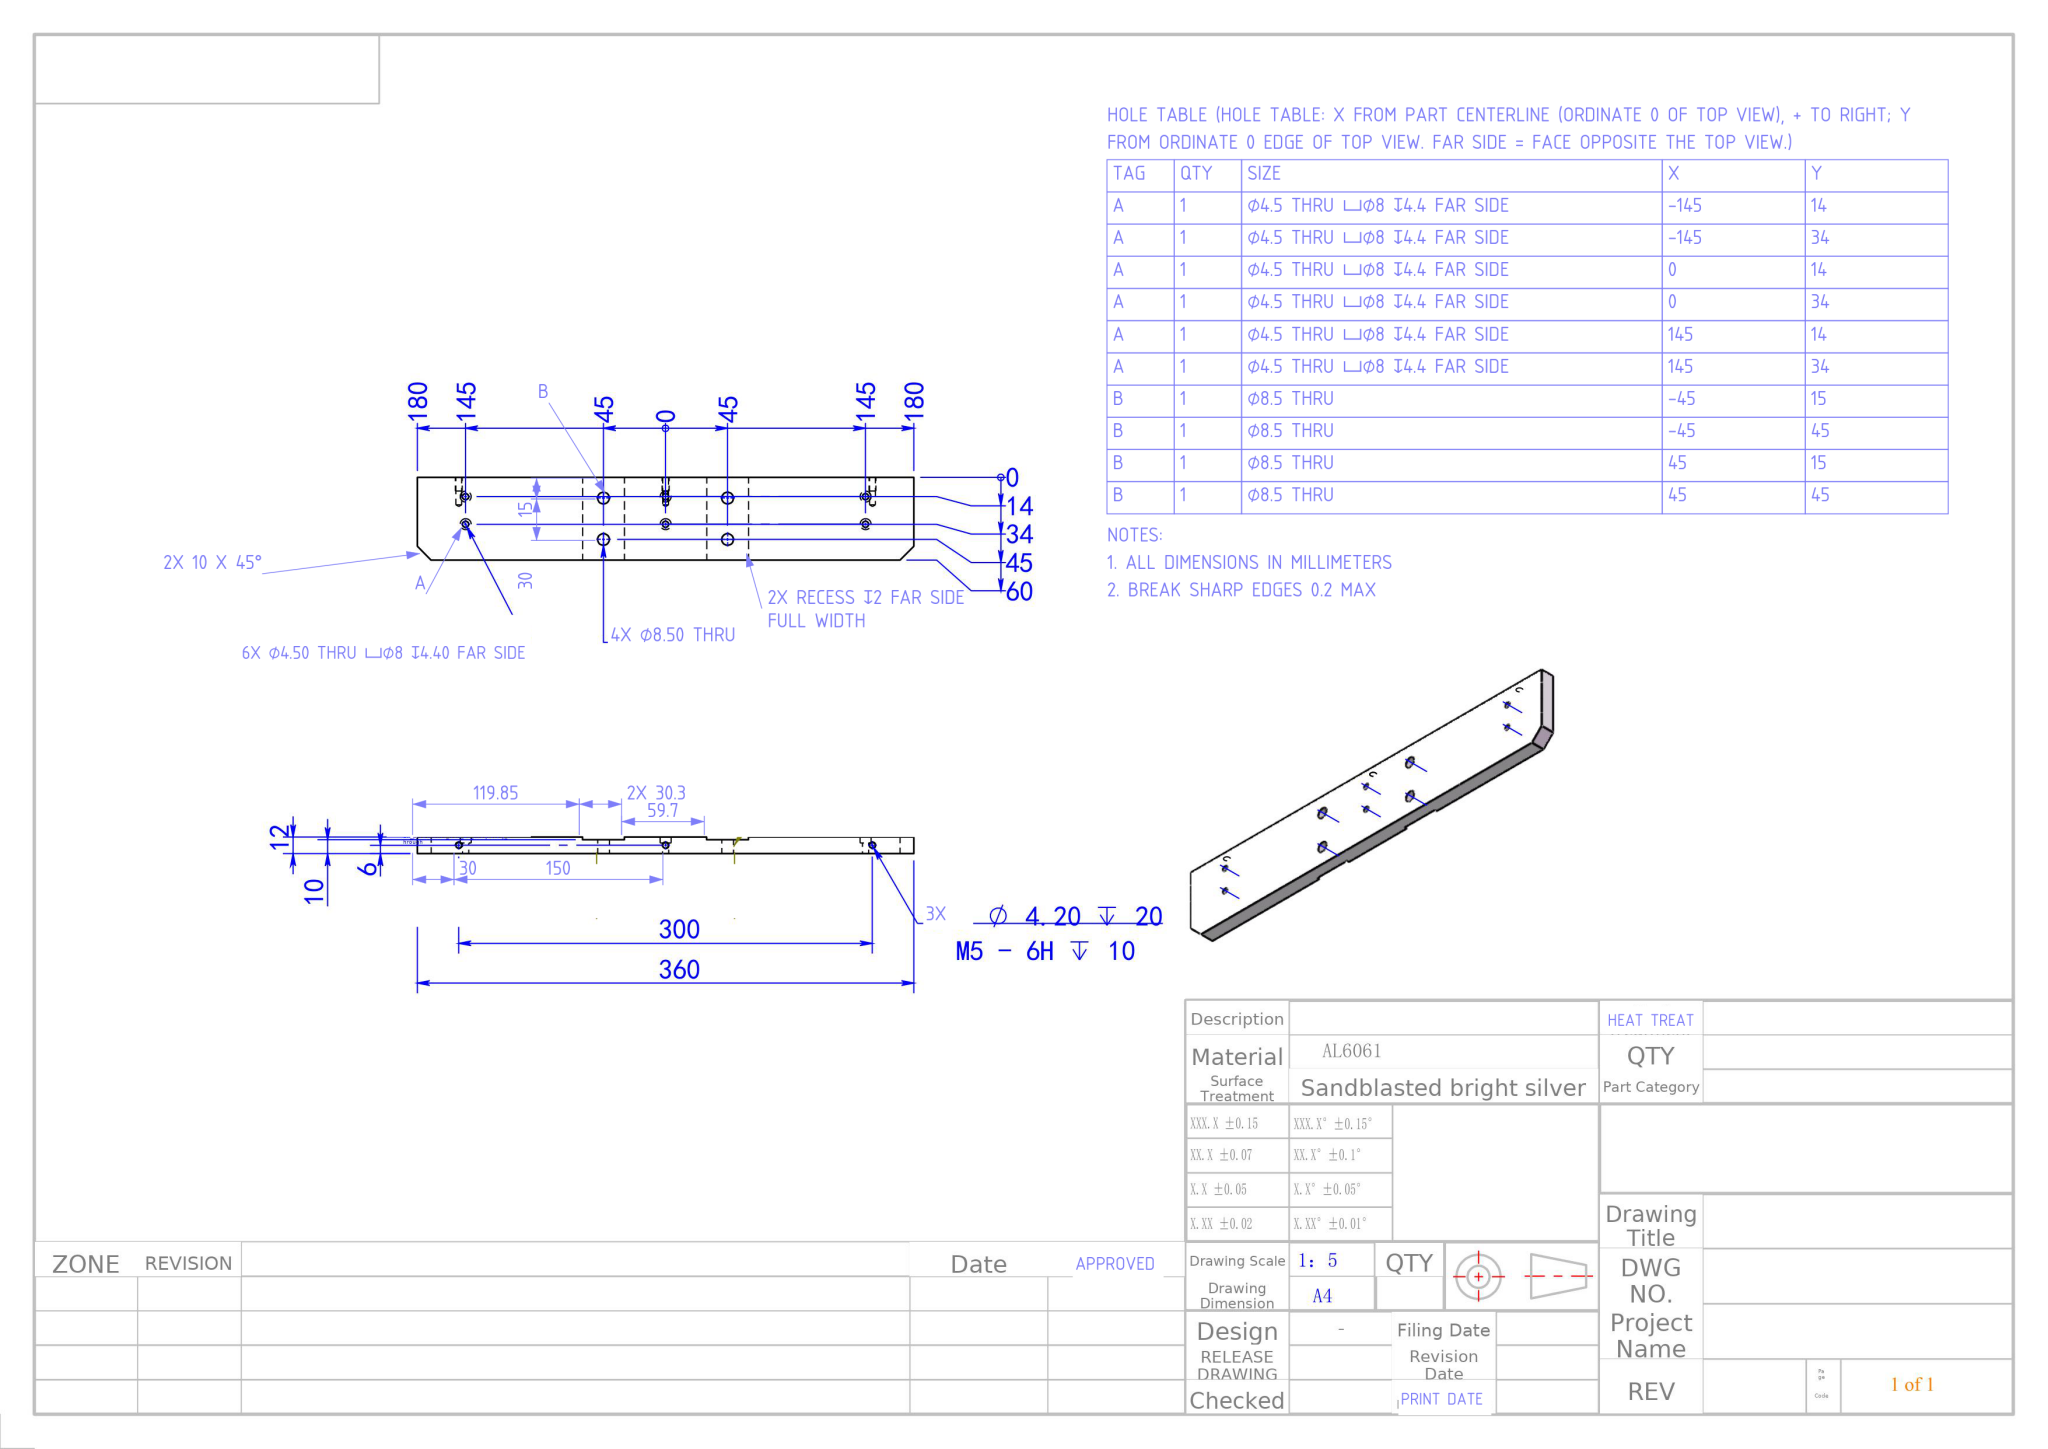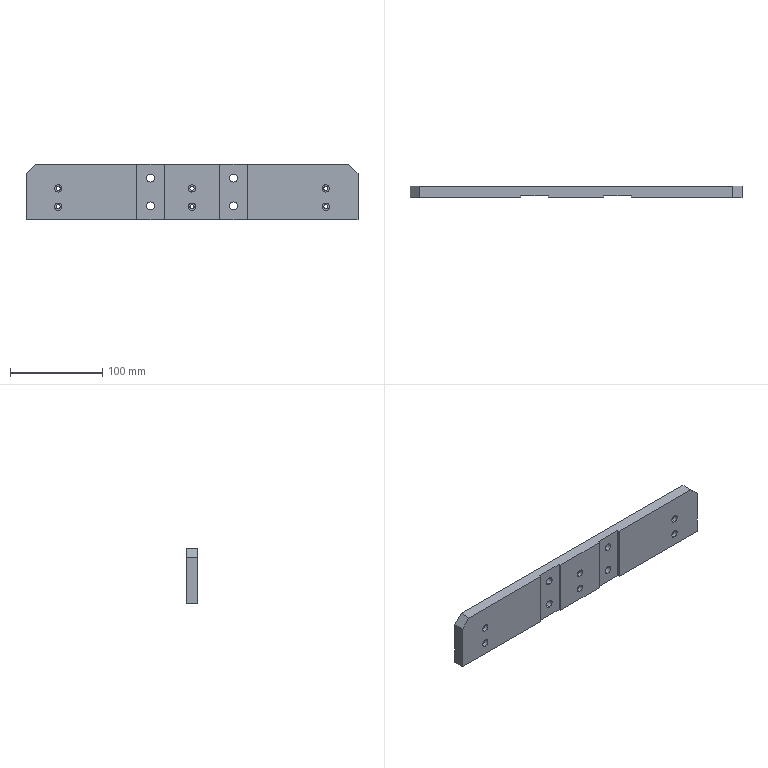Part | NX | mm | 1 solid | 69 faces | box 360 x 12 x 60 mm | volume 245615 mm3 | cylinder 40 | plane 23 | cone 6 | commonest cylinder face diameters 4.5 x12 8 x12 8.5 x8 4.2 x8